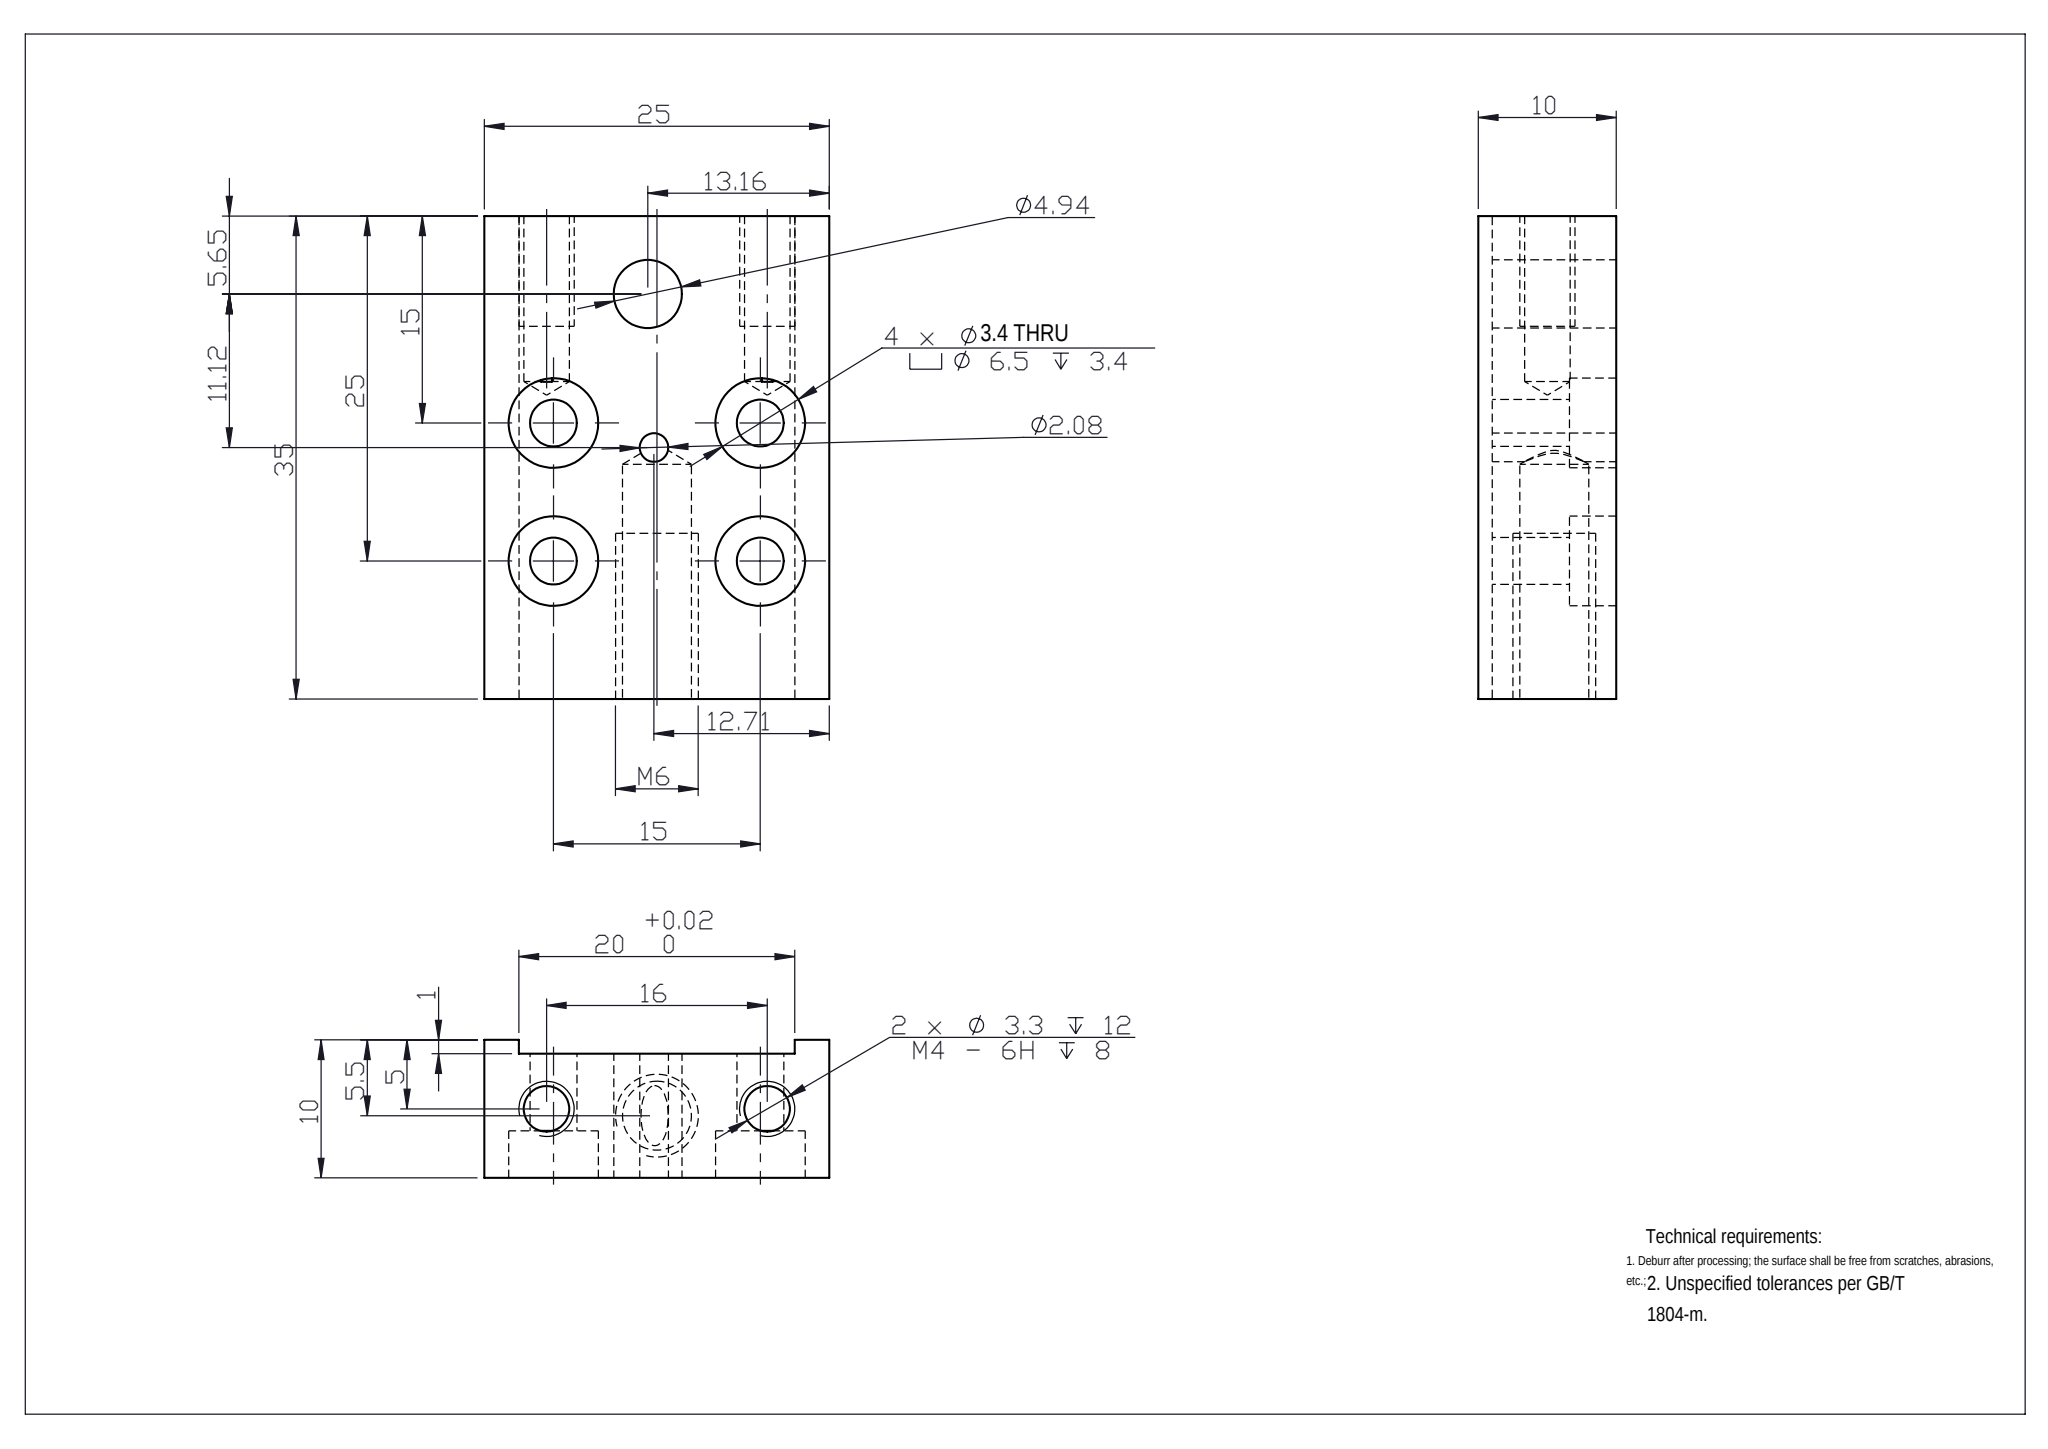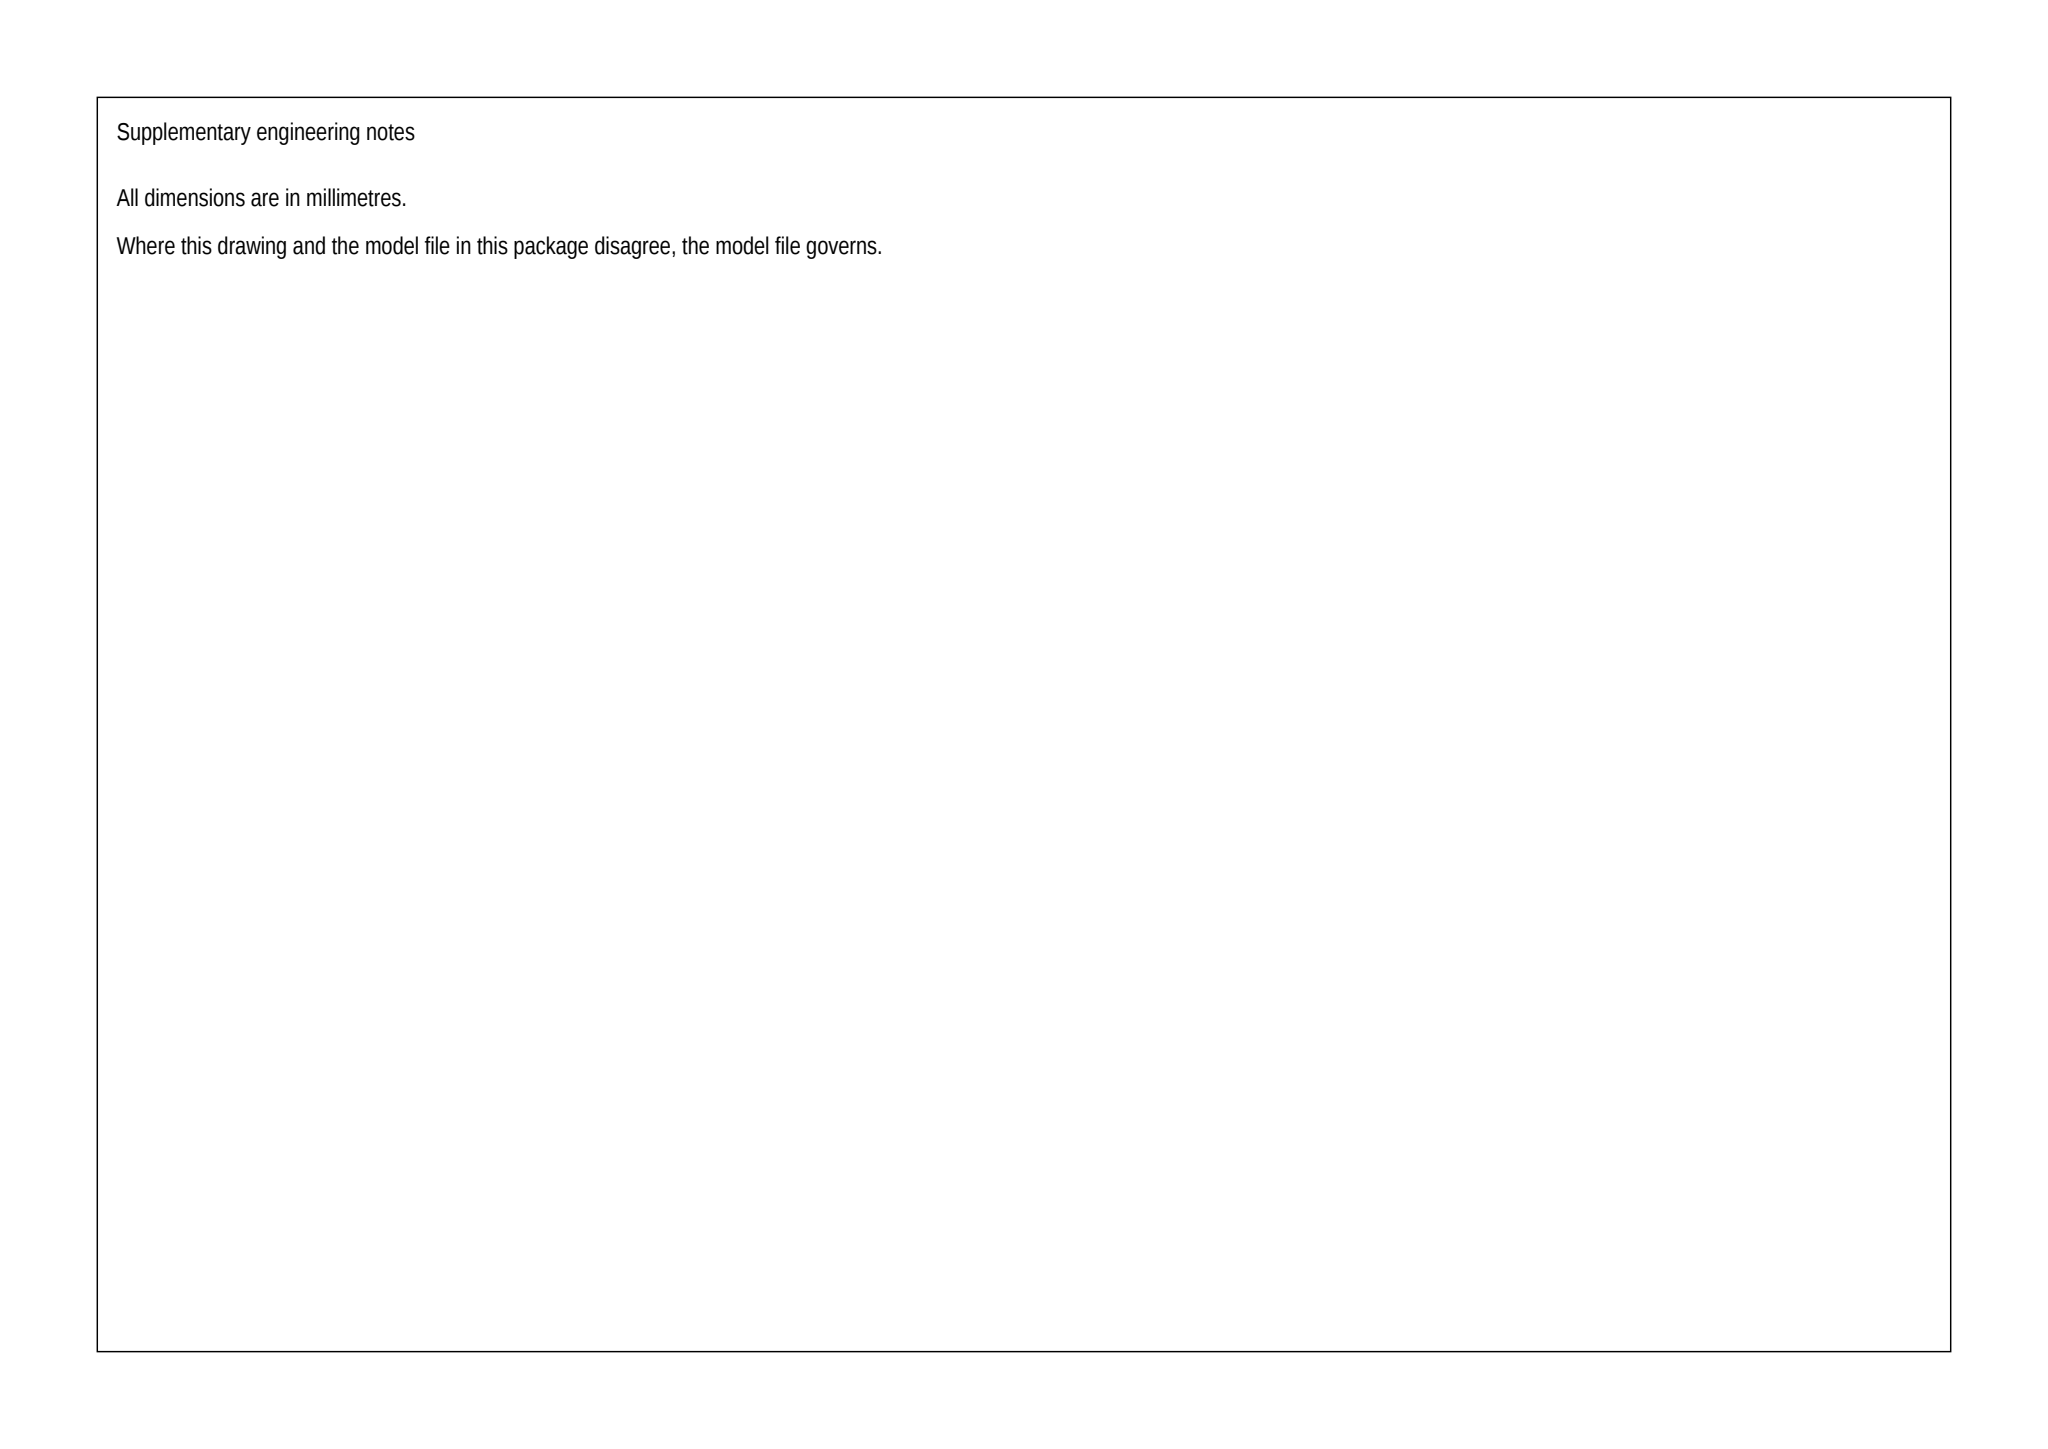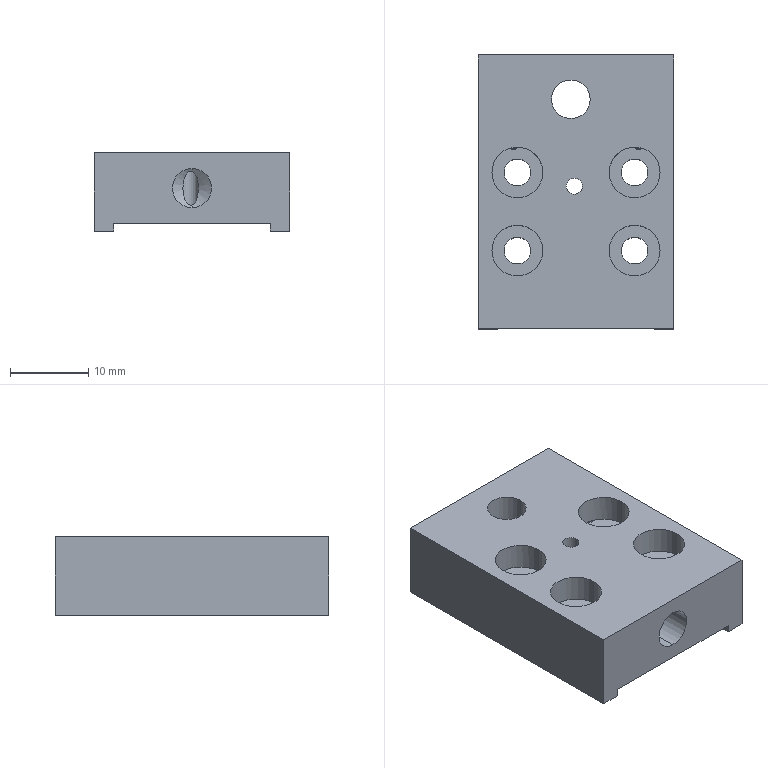Part | SolidWorks | mm | 1 solid | 46 faces | box 25 x 35 x 10 mm | volume 6641 mm3 | cylinder 26 | plane 14 | cone 6 | commonest cylinder face diameters 6.5 x8 3.4 x8 3.3 x4 4.943 x2 2.078 x2 5 x2
Drawing notes:
SLOT 20(+0.02/0) W x 1 DP x 35 FULL LG ON BACK FACE | from the solid: planes x=2.5 & x=22.5 (20 apart), floor z=1 vs lands z=0, bbox y=35
4X Ø3.4 THRU TO SLOT FLOOR, 5.6 DP BELOW CBORE Ø6.5 DP 3.4 | from the solid: cyl dia 3.4 axis z len 5.6 at (5,10)(5,20)(20,10)(20,20); cbore dia 6.5 len 3.4, z=6.6
Ø4.94 DP 9 FROM CBORED FACE TO SLOT FLOOR; 11.84 FR LH EDGE, 29.35 FR BTM EDGE | from the solid: cyl dia 4.943 axis z at (11.84,29.35), length 9.0, faces z=10 to z=1
Ø2.08 DP 9 TO SLOT FLOOR; 12.29 FR LH EDGE, 16.77 FR TOP EDGE | from the solid: cyl dia 2.078 axis z at (12.29,18.23), length 9.0; 35-18.23=16.77
M6 ON CL 12.5: TAP DRILL Ø5 DP 17 FROM BTM END FACE | from the solid: cyl dia 5.0 axis y at x=12.5 z=5.5, length 17.0; 118 deg cone ref dia 5
2X M4 CL 4.5 FR EA SIDE FACE, 5 FR SLOT FACE; FROM BTM END FACE | from the solid: cyl dia 3.3 axis y at x=4.5 & x=20.5, z=5.0, length 12.0; bbox x=25
build123d program:
from build123d import *

# Parameters (mm, degrees)
SKETCH1_W                                       = 25
SKETCH1_H                                       = 35
BOSS_EXTRUDE1_DEPTH                             = 10
M3_HEX_SOCKET_HEAD_CAP_SCREW_CBORE1_D           = 3.4
M3_HEX_SOCKET_HEAD_CAP_SCREW_CBORE1_CBORE_D     = 6.5
M3_HEX_SOCKET_HEAD_CAP_SCREW_CBORE1_CBORE_DEPTH = 3.4
SKETCH4_W                                       = 20
SKETCH4_H                                       = 35
CUT_EXTRUDE1_DEPTH                              = 1
M4_TAPPED_HOLE1_D                               = 3.3
M4_TAPPED_HOLE1_DEPTH                           = 12
M4_TAPPED_HOLE1_TIP                             = 0.9914
M6_TAPPED_HOLE1_D                               = 5
M6_TAPPED_HOLE1_DEPTH                           = 17
M6_TAPPED_HOLE1_TIP                             = 1.502
SKETCH10_R                                      = 2.472
SKETCH10_R_2                                    = 1.039
CUT_EXTRUDE2_DEPTH                              = 10


with BuildPart() as part:
    # Sketch1 → Boss-Extrude1 (new body)
    with BuildSketch(Plane.XY):
        with Locations((12.5, -17.5)):
            Rectangle(SKETCH1_W, SKETCH1_H)
    extrude(amount=BOSS_EXTRUDE1_DEPTH)

    # M3 Hex Socket Head Cap Screw CBORE1 (through all)
    with Locations(Plane.XY.offset(10)):
        with Locations((5, -15), (20, -15), (20, -25), (5, -25)):
            CounterBoreHole(M3_HEX_SOCKET_HEAD_CAP_SCREW_CBORE1_D / 2, M3_HEX_SOCKET_HEAD_CAP_SCREW_CBORE1_CBORE_D / 2, M3_HEX_SOCKET_HEAD_CAP_SCREW_CBORE1_CBORE_DEPTH)

    # Sketch4 → Cut-Extrude1 (cut)
    with BuildSketch(Plane(origin=(0, 0, 0), x_dir=(-1, 0, 0), z_dir=(0, 0, -1))):
        with Locations((-12.5, -17.5)):
            Rectangle(SKETCH4_W, SKETCH4_H)
    extrude(amount=-CUT_EXTRUDE1_DEPTH, mode=Mode.SUBTRACT)

    # M4 Tapped Hole1
    with Locations(Plane(origin=(0, 0, 0), x_dir=(1, 0, 0), z_dir=(0, 1, 0))):
        with Locations((20.5, -5), (4.5, -5)):
            Hole(M4_TAPPED_HOLE1_D / 2, depth=M4_TAPPED_HOLE1_DEPTH)
            with Locations((0, 0, -(M4_TAPPED_HOLE1_DEPTH + M4_TAPPED_HOLE1_TIP / 2))):  # 118° drill point
                Cone(0, M4_TAPPED_HOLE1_D / 2, M4_TAPPED_HOLE1_TIP, mode=Mode.SUBTRACT)

    # M6 Tapped Hole1
    with Locations(Plane(origin=(0, -35, 0), x_dir=(-1, 0, 0), z_dir=(0, -1, 0))):
        with Locations((-12.5, -5.5)):
            Hole(M6_TAPPED_HOLE1_D / 2, depth=M6_TAPPED_HOLE1_DEPTH)
            with Locations((0, 0, -(M6_TAPPED_HOLE1_DEPTH + M6_TAPPED_HOLE1_TIP / 2))):  # 118° drill point
                Cone(0, M6_TAPPED_HOLE1_D / 2, M6_TAPPED_HOLE1_TIP, mode=Mode.SUBTRACT)

    # Sketch10 → Cut-Extrude2 (cut)
    with BuildSketch(Plane.XY.offset(10)):
        with Locations((11.844, -5.651)):
            Circle(SKETCH10_R)
        with Locations((12.293, -16.773)):
            Circle(SKETCH10_R_2)
    extrude(amount=-CUT_EXTRUDE2_DEPTH, mode=Mode.SUBTRACT)


solid = part.part